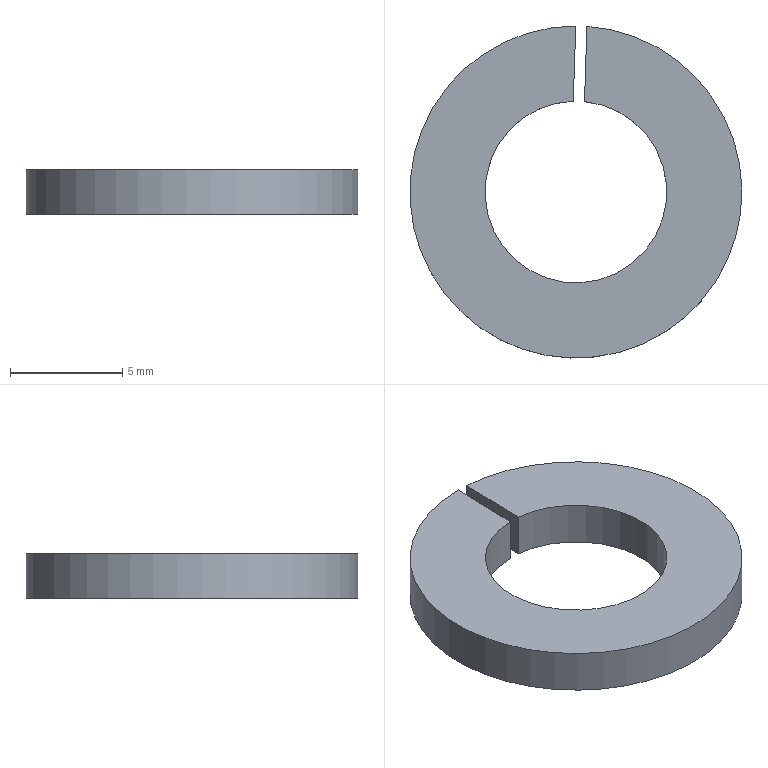Component | SolidWorks | ScrewM8-L35AndSpringWasherAssembly-2_SpringWasherTBN41-8(YIHEDA)-1 | 1 solid | 6 faces | box 14.8 x 14.8 x 2 mm | volume 238 mm3 | plane 4 | cylinder 2 | commonest cylinder face diameters 14.8 x1 8.1 x1
STEP:
#1=COLOUR_RGB('',0.7922,0.8196,0.9333);
#2=FILL_AREA_STYLE_COLOUR('',#1);
#3=FILL_AREA_STYLE('',(#2));
#4=SURFACE_STYLE_FILL_AREA(#3);
#5=SURFACE_SIDE_STYLE('',(#4));
#6=SURFACE_STYLE_USAGE(.BOTH.,#5);
#7=PRESENTATION_STYLE_ASSIGNMENT((#6));
#8=CARTESIAN_POINT('',(1.489,1.64,2.288));
#9=VERTEX_POINT('',#8);
#10=CARTESIAN_POINT('',(1.509,1.64,2.288));
#11=VERTEX_POINT('',#10);
#12=CARTESIAN_POINT('',(1.489,1.349,2.288));
#13=DIRECTION('',(0.,0.,1.));
#14=DIRECTION('',(-0.03295,-0.9995,0.));
#15=AXIS2_PLACEMENT_3D('',#12,#13,#14);
#16=CIRCLE('',#15,0.2913);
#17=EDGE_CURVE('',#9,#11,#16,.T.);
#18=ORIENTED_EDGE('',*,*,#17,.T.);
#19=CARTESIAN_POINT('',(1.509,1.64,2.366));
#20=VERTEX_POINT('',#19);
#21=CARTESIAN_POINT('',(1.509,1.64,2.366));
#22=DIRECTION('',(0.,0.,-1.));
#23=VECTOR('',#22,39.37);
#24=LINE('',#21,#23);
#25=EDGE_CURVE('',#20,#11,#24,.T.);
#26=ORIENTED_EDGE('',*,*,#25,.F.);
#27=CARTESIAN_POINT('',(1.489,1.64,2.366));
#28=VERTEX_POINT('',#27);
#29=CARTESIAN_POINT('',(1.489,1.349,2.366));
#30=DIRECTION('',(0.,0.,1.));
#31=DIRECTION('',(-0.03295,-0.9995,0.));
#32=AXIS2_PLACEMENT_3D('',#29,#30,#31);
#33=CIRCLE('',#32,0.2913);
#34=EDGE_CURVE('',#28,#20,#33,.T.);
#35=ORIENTED_EDGE('',*,*,#34,.F.);
#36=CARTESIAN_POINT('',(1.489,1.64,2.366));
#37=DIRECTION('',(0.,0.,-1.));
#38=VECTOR('',#37,39.37);
#39=LINE('',#36,#38);
#40=EDGE_CURVE('',#28,#9,#39,.T.);
#41=ORIENTED_EDGE('',*,*,#40,.T.);
#42=EDGE_LOOP('',(#18,#26,#35,#41));
#43=FACE_OUTER_BOUND('',#42,.T.);
#44=CARTESIAN_POINT('',(1.489,1.349,2.366));
#45=DIRECTION('',(0.,0.,1.));
#46=DIRECTION('',(0.03295,0.9995,0.));
#47=AXIS2_PLACEMENT_3D('',#44,#45,#46);
#48=CYLINDRICAL_SURFACE('',#47,0.2913);
#49=ADVANCED_FACE('',(#43),#48,.T.);
#50=ORIENTED_EDGE('',*,*,#34,.T.);
#51=CARTESIAN_POINT('',(1.504,1.508,2.366));
#52=VERTEX_POINT('',#51);
#53=CARTESIAN_POINT('',(1.509,1.64,2.366));
#54=DIRECTION('',(-0.03295,-0.9995,0.));
#55=VECTOR('',#54,39.37);
#56=LINE('',#53,#55);
#57=EDGE_CURVE('',#20,#52,#56,.T.);
#58=ORIENTED_EDGE('',*,*,#57,.T.);
#59=CARTESIAN_POINT('',(1.485,1.508,2.366));
#60=VERTEX_POINT('',#59);
#61=CARTESIAN_POINT('',(1.489,1.349,2.366));
#62=DIRECTION('',(0.,0.,1.));
#63=DIRECTION('',(-0.03295,-0.9995,0.));
#64=AXIS2_PLACEMENT_3D('',#61,#62,#63);
#65=CIRCLE('',#64,0.1594);
#66=EDGE_CURVE('',#60,#52,#65,.T.);
#67=ORIENTED_EDGE('',*,*,#66,.F.);
#68=CARTESIAN_POINT('',(1.485,1.508,2.366));
#69=DIRECTION('',(0.03295,0.9995,0.));
#70=VECTOR('',#69,39.37);
#71=LINE('',#68,#70);
#72=EDGE_CURVE('',#60,#28,#71,.T.);
#73=ORIENTED_EDGE('',*,*,#72,.T.);
#74=EDGE_LOOP('',(#50,#58,#67,#73));
#75=FACE_OUTER_BOUND('',#74,.T.);
#76=CARTESIAN_POINT('',(1.489,1.349,2.366));
#77=DIRECTION('',(0.,0.,1.));
#78=DIRECTION('',(-0.03295,-0.9995,0.));
#79=AXIS2_PLACEMENT_3D('',#76,#77,#78);
#80=PLANE('',#79);
#81=ADVANCED_FACE('',(#75),#80,.T.);
#82=CARTESIAN_POINT('',(1.504,1.508,2.288));
#83=VERTEX_POINT('',#82);
#84=CARTESIAN_POINT('',(1.509,1.64,2.288));
#85=DIRECTION('',(-0.03295,-0.9995,0.));
#86=VECTOR('',#85,39.37);
#87=LINE('',#84,#86);
#88=EDGE_CURVE('',#11,#83,#87,.T.);
#89=ORIENTED_EDGE('',*,*,#88,.T.);
#90=CARTESIAN_POINT('',(1.504,1.508,2.366));
#91=DIRECTION('',(0.,0.,-1.));
#92=VECTOR('',#91,39.37);
#93=LINE('',#90,#92);
#94=EDGE_CURVE('',#52,#83,#93,.T.);
#95=ORIENTED_EDGE('',*,*,#94,.F.);
#96=ORIENTED_EDGE('',*,*,#57,.F.);
#97=ORIENTED_EDGE('',*,*,#25,.T.);
#98=EDGE_LOOP('',(#89,#95,#96,#97));
#99=FACE_OUTER_BOUND('',#98,.T.);
#100=CARTESIAN_POINT('',(1.509,1.64,2.366));
#101=DIRECTION('',(0.9995,-0.03295,0.));
#102=DIRECTION('',(-0.03295,-0.9995,0.));
#103=AXIS2_PLACEMENT_3D('',#100,#101,#102);
#104=PLANE('',#103);
#105=ADVANCED_FACE('',(#99),#104,.F.);
#106=CARTESIAN_POINT('',(1.485,1.508,2.288));
#107=VERTEX_POINT('',#106);
#108=CARTESIAN_POINT('',(1.489,1.349,2.288));
#109=DIRECTION('',(0.,0.,1.));
#110=DIRECTION('',(-0.03295,-0.9995,0.));
#111=AXIS2_PLACEMENT_3D('',#108,#109,#110);
#112=CIRCLE('',#111,0.1594);
#113=EDGE_CURVE('',#107,#83,#112,.T.);
#114=ORIENTED_EDGE('',*,*,#113,.F.);
#115=CARTESIAN_POINT('',(1.485,1.508,2.366));
#116=DIRECTION('',(0.,0.,-1.));
#117=VECTOR('',#116,39.37);
#118=LINE('',#115,#117);
#119=EDGE_CURVE('',#60,#107,#118,.T.);
#120=ORIENTED_EDGE('',*,*,#119,.F.);
#121=ORIENTED_EDGE('',*,*,#66,.T.);
#122=ORIENTED_EDGE('',*,*,#94,.T.);
#123=EDGE_LOOP('',(#114,#120,#121,#122));
#124=FACE_OUTER_BOUND('',#123,.T.);
#125=CARTESIAN_POINT('',(1.489,1.349,2.366));
#126=DIRECTION('',(0.,0.,1.));
#127=DIRECTION('',(0.03295,0.9995,0.));
#128=AXIS2_PLACEMENT_3D('',#125,#126,#127);
#129=CYLINDRICAL_SURFACE('',#128,0.1594);
#130=ADVANCED_FACE('',(#124),#129,.F.);
#131=ORIENTED_EDGE('',*,*,#17,.F.);
#132=CARTESIAN_POINT('',(1.485,1.508,2.288));
#133=DIRECTION('',(0.03295,0.9995,0.));
#134=VECTOR('',#133,39.37);
#135=LINE('',#132,#134);
#136=EDGE_CURVE('',#107,#9,#135,.T.);
#137=ORIENTED_EDGE('',*,*,#136,.F.);
#138=ORIENTED_EDGE('',*,*,#113,.T.);
#139=ORIENTED_EDGE('',*,*,#88,.F.);
#140=EDGE_LOOP('',(#131,#137,#138,#139));
#141=FACE_OUTER_BOUND('',#140,.T.);
#142=CARTESIAN_POINT('',(1.489,1.349,2.288));
#143=DIRECTION('',(0.,0.,1.));
#144=DIRECTION('',(-0.03295,-0.9995,0.));
#145=AXIS2_PLACEMENT_3D('',#142,#143,#144);
#146=PLANE('',#145);
#147=ADVANCED_FACE('',(#141),#146,.F.);
#148=ORIENTED_EDGE('',*,*,#136,.T.);
#149=ORIENTED_EDGE('',*,*,#40,.F.);
#150=ORIENTED_EDGE('',*,*,#72,.F.);
#151=ORIENTED_EDGE('',*,*,#119,.T.);
#152=EDGE_LOOP('',(#148,#149,#150,#151));
#153=FACE_OUTER_BOUND('',#152,.T.);
#154=CARTESIAN_POINT('',(1.485,1.508,2.366));
#155=DIRECTION('',(-0.9995,0.03295,0.));
#156=DIRECTION('',(0.,0.,-1.));
#157=AXIS2_PLACEMENT_3D('',#154,#155,#156);
#158=PLANE('',#157);
#159=ADVANCED_FACE('',(#153),#158,.F.);
#160=CLOSED_SHELL('',(#49,#81,#105,#130,#147,#159));
#161=MANIFOLD_SOLID_BREP('',#160);
#162=STYLED_ITEM('',(#7),#161);
#163=PRESENTATION_LAYER_ASSIGNMENT('','',(#162));
#164=(LENGTH_UNIT()NAMED_UNIT(*)SI_UNIT($,.METRE.));
#165=LENGTH_MEASURE_WITH_UNIT(LENGTH_MEASURE(0.0254),#164);
#166=DIMENSIONAL_EXPONENTS(1.,0.,0.,0.,0.,0.,0.);
#167=(CONVERSION_BASED_UNIT('',#165)LENGTH_UNIT()NAMED_UNIT(#166));
#168=UNCERTAINTY_MEASURE_WITH_UNIT(LENGTH_MEASURE(0.00001),#167,'','');
#169=(NAMED_UNIT(*)PLANE_ANGLE_UNIT()SI_UNIT($,.RADIAN.));
#170=(NAMED_UNIT(*)SI_UNIT($,.STERADIAN.)SOLID_ANGLE_UNIT());
#171=(GEOMETRIC_REPRESENTATION_CONTEXT(3)GLOBAL_UNCERTAINTY_ASSIGNED_CONTEXT((#168))GLOBAL_UNIT_ASSIGNED_CONTEXT((#167,#169,#170))REPRESENTATION_CONTEXT('',''));
#172=MECHANICAL_DESIGN_GEOMETRIC_PRESENTATION_REPRESENTATION('',(#162),#171);
#173=CARTESIAN_POINT('',(0.,0.,0.));
#174=DIRECTION('',(0.,0.,1.));
#175=DIRECTION('',(1.,0.,0.));
#176=AXIS2_PLACEMENT_3D('',#173,#174,#175);
#177=(LENGTH_UNIT()NAMED_UNIT(*)SI_UNIT($,.METRE.));
#178=LENGTH_MEASURE_WITH_UNIT(LENGTH_MEASURE(0.0254),#177);
#179=DIMENSIONAL_EXPONENTS(1.,0.,0.,0.,0.,0.,0.);
#180=(CONVERSION_BASED_UNIT('',#178)LENGTH_UNIT()NAMED_UNIT(#179));
#181=UNCERTAINTY_MEASURE_WITH_UNIT(LENGTH_MEASURE(0.00001),#180,'','');
#182=(NAMED_UNIT(*)PLANE_ANGLE_UNIT()SI_UNIT($,.RADIAN.));
#183=(NAMED_UNIT(*)SI_UNIT($,.STERADIAN.)SOLID_ANGLE_UNIT());
#184=(GEOMETRIC_REPRESENTATION_CONTEXT(3)GLOBAL_UNCERTAINTY_ASSIGNED_CONTEXT((#181))GLOBAL_UNIT_ASSIGNED_CONTEXT((#180,#182,#183))REPRESENTATION_CONTEXT('',''));
#185=ADVANCED_BREP_SHAPE_REPRESENTATION('',(#161,#176),#184);